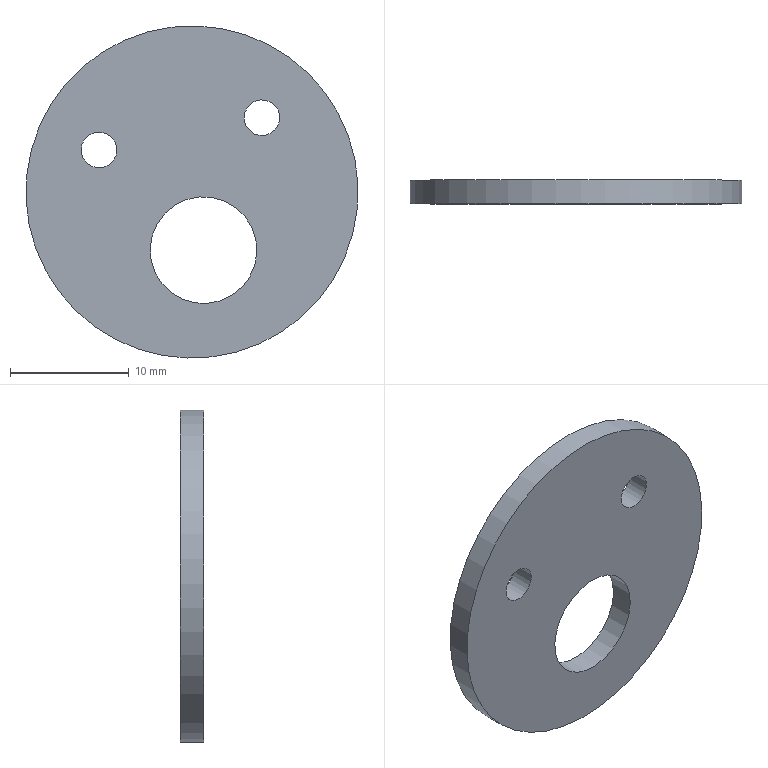Component | NX | ECCENTRIC_SIDE_PLATE_2 | 1 solid | 6 faces | box 28 x 2 x 28 mm | volume 1076 mm3 | cylinder 4 | plane 2 | commonest cylinder face diameters 3 x2 28 x1 9 x1
STEP:
#1=CARTESIAN_POINT('',(0.,0.,0.));
#2=DIRECTION('',(0.,0.,1.));
#3=DIRECTION('',(1.,0.,0.));
#4=AXIS2_PLACEMENT_3D('',#1,#2,#3);
#5=CARTESIAN_POINT('',(49.953,-62.5,29.378));
#6=VERTEX_POINT('',#5);
#7=CARTESIAN_POINT('',(51.424,-62.5,29.669));
#8=DIRECTION('',(0.,1.,0.));
#9=DIRECTION('',(-0.9809,0.,-0.1943));
#10=AXIS2_PLACEMENT_3D('',#7,#8,#9);
#11=CIRCLE('',#10,1.5);
#12=CARTESIAN_POINT('',(45.529,-62.5,23.405));
#13=DIRECTION('',(0.,-1.,0.));
#14=DIRECTION('',(-0.9809,0.,-0.1943));
#15=AXIS2_PLACEMENT_3D('',#12,#13,#14);
#16=PLANE('',#15);
#17=CARTESIAN_POINT('',(-5.5,-5.));
#18=CARTESIAN_POINT('',(-5.5,-7.598));
#19=CARTESIAN_POINT('',(-7.75,-6.299));
#20=CARTESIAN_POINT('',(-10.,-5.));
#21=CARTESIAN_POINT('',(-7.75,-3.701));
#22=CARTESIAN_POINT('',(-5.5,-2.402));
#23=CARTESIAN_POINT('',(-5.5,-5.));
#24=(BOUNDED_CURVE()B_SPLINE_CURVE(2,(#17,#18,#19,#20,#21,#22,#23),.UNSPECIFIED.,.T.,.F.)B_SPLINE_CURVE_WITH_KNOTS((1,2,2,2,2,1),(-2.094,0.,2.094,4.189,6.283,8.378),.UNSPECIFIED.)CURVE()GEOMETRIC_REPRESENTATION_ITEM()RATIONAL_B_SPLINE_CURVE((1.,0.5,1.,0.5,1.,0.5,1.))REPRESENTATION_ITEM(''));
#25=(GEOMETRIC_REPRESENTATION_CONTEXT(2)PARAMETRIC_REPRESENTATION_CONTEXT()REPRESENTATION_CONTEXT('',''));
#26=DEFINITIONAL_REPRESENTATION('',(#24),#25);
#27=PCURVE('',#16,#26);
#28=CARTESIAN_POINT('',(51.424,-42.5,29.669));
#29=DIRECTION('',(0.,-1.,0.));
#30=DIRECTION('',(-0.9809,0.,-0.1943));
#31=AXIS2_PLACEMENT_3D('',#28,#29,#30);
#32=CYLINDRICAL_SURFACE('',#31,1.5);
#33=CARTESIAN_POINT('',(6.283,20.));
#34=DIRECTION('',(-1.,0.));
#35=VECTOR('',#34,1.);
#36=LINE('',#33,#35);
#37=(GEOMETRIC_REPRESENTATION_CONTEXT(2)PARAMETRIC_REPRESENTATION_CONTEXT()REPRESENTATION_CONTEXT('',''));
#38=DEFINITIONAL_REPRESENTATION('',(#36),#37);
#39=PCURVE('',#32,#38);
#40=SURFACE_CURVE('',#11,(#27,#39),.PCURVE_S1.);
#41=EDGE_CURVE('',#6,#6,#40,.T.);
#42=ORIENTED_EDGE('',*,*,#41,.T.);
#43=EDGE_LOOP('',(#42));
#44=FACE_BOUND('',#43,.T.);
#45=CARTESIAN_POINT('',(42.086,-62.5,17.626));
#46=VERTEX_POINT('',#45);
#47=CARTESIAN_POINT('',(46.5,-62.5,18.5));
#48=DIRECTION('',(0.,1.,0.));
#49=DIRECTION('',(-0.9809,0.,-0.1943));
#50=AXIS2_PLACEMENT_3D('',#47,#48,#49);
#51=CIRCLE('',#50,4.5);
#52=CARTESIAN_POINT('',(4.5,5.));
#53=CARTESIAN_POINT('',(4.5,-2.794));
#54=CARTESIAN_POINT('',(-2.25,1.103));
#55=CARTESIAN_POINT('',(-9.,5.));
#56=CARTESIAN_POINT('',(-2.25,8.897));
#57=CARTESIAN_POINT('',(4.5,12.794));
#58=CARTESIAN_POINT('',(4.5,5.));
#59=(BOUNDED_CURVE()B_SPLINE_CURVE(2,(#52,#53,#54,#55,#56,#57,#58),.UNSPECIFIED.,.T.,.F.)B_SPLINE_CURVE_WITH_KNOTS((1,2,2,2,2,1),(-2.094,0.,2.094,4.189,6.283,8.378),.UNSPECIFIED.)CURVE()GEOMETRIC_REPRESENTATION_ITEM()RATIONAL_B_SPLINE_CURVE((1.,0.5,1.,0.5,1.,0.5,1.))REPRESENTATION_ITEM(''));
#60=(GEOMETRIC_REPRESENTATION_CONTEXT(2)PARAMETRIC_REPRESENTATION_CONTEXT()REPRESENTATION_CONTEXT('',''));
#61=DEFINITIONAL_REPRESENTATION('',(#59),#60);
#62=PCURVE('',#16,#61);
#63=CARTESIAN_POINT('',(46.5,-42.5,18.5));
#64=DIRECTION('',(0.,-1.,0.));
#65=DIRECTION('',(-0.9809,0.,-0.1943));
#66=AXIS2_PLACEMENT_3D('',#63,#64,#65);
#67=CYLINDRICAL_SURFACE('',#66,4.5);
#68=CARTESIAN_POINT('',(6.283,20.));
#69=DIRECTION('',(-1.,0.));
#70=VECTOR('',#69,1.);
#71=LINE('',#68,#70);
#72=(GEOMETRIC_REPRESENTATION_CONTEXT(2)PARAMETRIC_REPRESENTATION_CONTEXT()REPRESENTATION_CONTEXT('',''));
#73=DEFINITIONAL_REPRESENTATION('',(#71),#72);
#74=PCURVE('',#67,#73);
#75=SURFACE_CURVE('',#51,(#62,#74),.PCURVE_S1.);
#76=EDGE_CURVE('',#46,#46,#75,.T.);
#77=ORIENTED_EDGE('',*,*,#76,.T.);
#78=EDGE_LOOP('',(#77));
#79=FACE_BOUND('',#78,.T.);
#80=CARTESIAN_POINT('',(31.795,-62.5,20.685));
#81=VERTEX_POINT('',#80);
#82=CARTESIAN_POINT('',(45.529,-62.5,23.405));
#83=DIRECTION('',(0.,1.,0.));
#84=DIRECTION('',(-0.9809,0.,-0.1943));
#85=AXIS2_PLACEMENT_3D('',#82,#83,#84);
#86=CIRCLE('',#85,14.);
#87=CARTESIAN_POINT('',(14.,0.));
#88=CARTESIAN_POINT('',(14.,-24.249));
#89=CARTESIAN_POINT('',(-7.,-12.124));
#90=CARTESIAN_POINT('',(-28.,-0.));
#91=CARTESIAN_POINT('',(-7.,12.124));
#92=CARTESIAN_POINT('',(14.,24.249));
#93=CARTESIAN_POINT('',(14.,0.));
#94=(BOUNDED_CURVE()B_SPLINE_CURVE(2,(#87,#88,#89,#90,#91,#92,#93),.UNSPECIFIED.,.T.,.F.)B_SPLINE_CURVE_WITH_KNOTS((1,2,2,2,2,1),(-2.094,0.,2.094,4.189,6.283,8.378),.UNSPECIFIED.)CURVE()GEOMETRIC_REPRESENTATION_ITEM()RATIONAL_B_SPLINE_CURVE((1.,0.5,1.,0.5,1.,0.5,1.))REPRESENTATION_ITEM(''));
#95=(GEOMETRIC_REPRESENTATION_CONTEXT(2)PARAMETRIC_REPRESENTATION_CONTEXT()REPRESENTATION_CONTEXT('',''));
#96=DEFINITIONAL_REPRESENTATION('',(#94),#95);
#97=PCURVE('',#16,#96);
#98=CARTESIAN_POINT('',(45.529,-60.5,23.405));
#99=DIRECTION('',(0.,-1.,0.));
#100=DIRECTION('',(-0.9809,0.,-0.1943));
#101=AXIS2_PLACEMENT_3D('',#98,#99,#100);
#102=CYLINDRICAL_SURFACE('',#101,14.);
#103=CARTESIAN_POINT('',(6.283,2.));
#104=DIRECTION('',(-1.,0.));
#105=VECTOR('',#104,1.);
#106=LINE('',#103,#105);
#107=(GEOMETRIC_REPRESENTATION_CONTEXT(2)PARAMETRIC_REPRESENTATION_CONTEXT()REPRESENTATION_CONTEXT('',''));
#108=DEFINITIONAL_REPRESENTATION('',(#106),#107);
#109=PCURVE('',#102,#108);
#110=SURFACE_CURVE('',#86,(#97,#109),.PCURVE_S1.);
#111=EDGE_CURVE('',#81,#81,#110,.T.);
#112=ORIENTED_EDGE('',*,*,#111,.F.);
#113=EDGE_LOOP('',(#112));
#114=FACE_BOUND('',#113,.T.);
#115=CARTESIAN_POINT('',(39.162,-62.5,27.241));
#116=VERTEX_POINT('',#115);
#117=CARTESIAN_POINT('',(37.691,-62.5,26.95));
#118=DIRECTION('',(0.,-1.,0.));
#119=DIRECTION('',(0.9809,0.,0.1943));
#120=AXIS2_PLACEMENT_3D('',#117,#118,#119);
#121=CIRCLE('',#120,1.5);
#122=CARTESIAN_POINT('',(7.,-5.));
#123=DIRECTION('',(-1.,0.));
#124=AXIS2_PLACEMENT_2D('',#122,#123);
#125=CIRCLE('',#124,1.5);
#126=(GEOMETRIC_REPRESENTATION_CONTEXT(2)PARAMETRIC_REPRESENTATION_CONTEXT()REPRESENTATION_CONTEXT('',''));
#127=DEFINITIONAL_REPRESENTATION('',(#125),#126);
#128=PCURVE('',#16,#127);
#129=CARTESIAN_POINT('',(37.691,-42.5,26.95));
#130=DIRECTION('',(0.,-1.,0.));
#131=DIRECTION('',(-0.9809,0.,-0.1943));
#132=AXIS2_PLACEMENT_3D('',#129,#130,#131);
#133=CYLINDRICAL_SURFACE('',#132,1.5);
#134=CARTESIAN_POINT('',(3.142,20.));
#135=DIRECTION('',(1.,0.));
#136=VECTOR('',#135,1.);
#137=LINE('',#134,#136);
#138=(GEOMETRIC_REPRESENTATION_CONTEXT(2)PARAMETRIC_REPRESENTATION_CONTEXT()REPRESENTATION_CONTEXT('',''));
#139=DEFINITIONAL_REPRESENTATION('',(#137),#138);
#140=PCURVE('',#133,#139);
#141=SURFACE_CURVE('',#121,(#128,#140),.PCURVE_S1.);
#142=EDGE_CURVE('',#116,#116,#141,.T.);
#143=ORIENTED_EDGE('',*,*,#142,.F.);
#144=EDGE_LOOP('',(#143));
#145=FACE_BOUND('',#144,.T.);
#146=ADVANCED_FACE('',(#44,#79,#114,#145),#16,.T.);
#147=CARTESIAN_POINT('',(52.895,-60.5,29.961));
#148=VERTEX_POINT('',#147);
#149=CARTESIAN_POINT('',(49.953,-60.5,29.378));
#150=VERTEX_POINT('',#149);
#151=CARTESIAN_POINT('',(51.424,-60.5,29.669));
#152=DIRECTION('',(0.,-1.,0.));
#153=DIRECTION('',(0.9809,0.,0.1943));
#154=AXIS2_PLACEMENT_3D('',#151,#152,#153);
#155=CIRCLE('',#154,1.5);
#156=CARTESIAN_POINT('',(45.529,-60.5,23.405));
#157=DIRECTION('',(0.,1.,0.));
#158=DIRECTION('',(0.9809,0.,0.1943));
#159=AXIS2_PLACEMENT_3D('',#156,#157,#158);
#160=PLANE('',#159);
#161=CARTESIAN_POINT('',(8.5,-5.));
#162=CARTESIAN_POINT('',(8.5,-7.598));
#163=CARTESIAN_POINT('',(6.25,-6.299));
#164=CARTESIAN_POINT('',(4.,-5.));
#165=CARTESIAN_POINT('',(6.25,-3.701));
#166=CARTESIAN_POINT('',(8.5,-2.402));
#167=CARTESIAN_POINT('',(8.5,-5.));
#168=(BOUNDED_CURVE()B_SPLINE_CURVE(2,(#161,#162,#163,#164,#165,#166,#167),.UNSPECIFIED.,.T.,.F.)B_SPLINE_CURVE_WITH_KNOTS((1,2,2,2,2,1),(-2.094,0.,2.094,4.189,6.283,8.378),.UNSPECIFIED.)CURVE()GEOMETRIC_REPRESENTATION_ITEM()RATIONAL_B_SPLINE_CURVE((1.,0.5,1.,0.5,1.,0.5,1.))REPRESENTATION_ITEM(''));
#169=(GEOMETRIC_REPRESENTATION_CONTEXT(2)PARAMETRIC_REPRESENTATION_CONTEXT()REPRESENTATION_CONTEXT('',''));
#170=DEFINITIONAL_REPRESENTATION('',(#168),#169);
#171=PCURVE('',#160,#170);
#172=CARTESIAN_POINT('',(3.142,18.));
#173=DIRECTION('',(1.,0.));
#174=VECTOR('',#173,1.);
#175=LINE('',#172,#174);
#176=(GEOMETRIC_REPRESENTATION_CONTEXT(2)PARAMETRIC_REPRESENTATION_CONTEXT()REPRESENTATION_CONTEXT('',''));
#177=DEFINITIONAL_REPRESENTATION('',(#175),#176);
#178=PCURVE('',#32,#177);
#179=SURFACE_CURVE('',#155,(#171,#178),.PCURVE_S1.);
#180=EDGE_CURVE('',#148,#150,#179,.T.);
#181=ORIENTED_EDGE('',*,*,#180,.T.);
#182=CARTESIAN_POINT('',(51.424,-60.5,29.669));
#183=DIRECTION('',(0.,-1.,0.));
#184=DIRECTION('',(0.9809,0.,0.1943));
#185=AXIS2_PLACEMENT_3D('',#182,#183,#184);
#186=CIRCLE('',#185,1.5);
#187=CARTESIAN_POINT('',(8.5,-5.));
#188=CARTESIAN_POINT('',(8.5,-7.598));
#189=CARTESIAN_POINT('',(6.25,-6.299));
#190=CARTESIAN_POINT('',(4.,-5.));
#191=CARTESIAN_POINT('',(6.25,-3.701));
#192=CARTESIAN_POINT('',(8.5,-2.402));
#193=CARTESIAN_POINT('',(8.5,-5.));
#194=(BOUNDED_CURVE()B_SPLINE_CURVE(2,(#187,#188,#189,#190,#191,#192,#193),.UNSPECIFIED.,.T.,.F.)B_SPLINE_CURVE_WITH_KNOTS((1,2,2,2,2,1),(-2.094,0.,2.094,4.189,6.283,8.378),.UNSPECIFIED.)CURVE()GEOMETRIC_REPRESENTATION_ITEM()RATIONAL_B_SPLINE_CURVE((1.,0.5,1.,0.5,1.,0.5,1.))REPRESENTATION_ITEM(''));
#195=(GEOMETRIC_REPRESENTATION_CONTEXT(2)PARAMETRIC_REPRESENTATION_CONTEXT()REPRESENTATION_CONTEXT('',''));
#196=DEFINITIONAL_REPRESENTATION('',(#194),#195);
#197=PCURVE('',#160,#196);
#198=CARTESIAN_POINT('',(-3.142,18.));
#199=DIRECTION('',(1.,0.));
#200=VECTOR('',#199,1.);
#201=LINE('',#198,#200);
#202=(GEOMETRIC_REPRESENTATION_CONTEXT(2)PARAMETRIC_REPRESENTATION_CONTEXT()REPRESENTATION_CONTEXT('',''));
#203=DEFINITIONAL_REPRESENTATION('',(#201),#202);
#204=PCURVE('',#32,#203);
#205=SURFACE_CURVE('',#186,(#197,#204),.PCURVE_S1.);
#206=EDGE_CURVE('',#150,#148,#205,.T.);
#207=ORIENTED_EDGE('',*,*,#206,.T.);
#208=EDGE_LOOP('',(#181,#207));
#209=FACE_BOUND('',#208,.T.);
#210=CARTESIAN_POINT('',(50.914,-60.5,19.374));
#211=VERTEX_POINT('',#210);
#212=CARTESIAN_POINT('',(42.086,-60.5,17.626));
#213=VERTEX_POINT('',#212);
#214=CARTESIAN_POINT('',(46.5,-60.5,18.5));
#215=DIRECTION('',(0.,-1.,0.));
#216=DIRECTION('',(0.9809,0.,0.1943));
#217=AXIS2_PLACEMENT_3D('',#214,#215,#216);
#218=CIRCLE('',#217,4.5);
#219=CARTESIAN_POINT('',(4.5,5.));
#220=CARTESIAN_POINT('',(4.5,-2.794));
#221=CARTESIAN_POINT('',(-2.25,1.103));
#222=CARTESIAN_POINT('',(-9.,5.));
#223=CARTESIAN_POINT('',(-2.25,8.897));
#224=CARTESIAN_POINT('',(4.5,12.794));
#225=CARTESIAN_POINT('',(4.5,5.));
#226=(BOUNDED_CURVE()B_SPLINE_CURVE(2,(#219,#220,#221,#222,#223,#224,#225),.UNSPECIFIED.,.T.,.F.)B_SPLINE_CURVE_WITH_KNOTS((1,2,2,2,2,1),(-2.094,0.,2.094,4.189,6.283,8.378),.UNSPECIFIED.)CURVE()GEOMETRIC_REPRESENTATION_ITEM()RATIONAL_B_SPLINE_CURVE((1.,0.5,1.,0.5,1.,0.5,1.))REPRESENTATION_ITEM(''));
#227=(GEOMETRIC_REPRESENTATION_CONTEXT(2)PARAMETRIC_REPRESENTATION_CONTEXT()REPRESENTATION_CONTEXT('',''));
#228=DEFINITIONAL_REPRESENTATION('',(#226),#227);
#229=PCURVE('',#160,#228);
#230=CARTESIAN_POINT('',(3.142,18.));
#231=DIRECTION('',(1.,0.));
#232=VECTOR('',#231,1.);
#233=LINE('',#230,#232);
#234=(GEOMETRIC_REPRESENTATION_CONTEXT(2)PARAMETRIC_REPRESENTATION_CONTEXT()REPRESENTATION_CONTEXT('',''));
#235=DEFINITIONAL_REPRESENTATION('',(#233),#234);
#236=PCURVE('',#67,#235);
#237=SURFACE_CURVE('',#218,(#229,#236),.PCURVE_S1.);
#238=EDGE_CURVE('',#211,#213,#237,.T.);
#239=ORIENTED_EDGE('',*,*,#238,.T.);
#240=CARTESIAN_POINT('',(46.5,-60.5,18.5));
#241=DIRECTION('',(0.,-1.,0.));
#242=DIRECTION('',(0.9809,0.,0.1943));
#243=AXIS2_PLACEMENT_3D('',#240,#241,#242);
#244=CIRCLE('',#243,4.5);
#245=CARTESIAN_POINT('',(4.5,5.));
#246=CARTESIAN_POINT('',(4.5,-2.794));
#247=CARTESIAN_POINT('',(-2.25,1.103));
#248=CARTESIAN_POINT('',(-9.,5.));
#249=CARTESIAN_POINT('',(-2.25,8.897));
#250=CARTESIAN_POINT('',(4.5,12.794));
#251=CARTESIAN_POINT('',(4.5,5.));
#252=(BOUNDED_CURVE()B_SPLINE_CURVE(2,(#245,#246,#247,#248,#249,#250,#251),.UNSPECIFIED.,.T.,.F.)B_SPLINE_CURVE_WITH_KNOTS((1,2,2,2,2,1),(-2.094,0.,2.094,4.189,6.283,8.378),.UNSPECIFIED.)CURVE()GEOMETRIC_REPRESENTATION_ITEM()RATIONAL_B_SPLINE_CURVE((1.,0.5,1.,0.5,1.,0.5,1.))REPRESENTATION_ITEM(''));
#253=(GEOMETRIC_REPRESENTATION_CONTEXT(2)PARAMETRIC_REPRESENTATION_CONTEXT()REPRESENTATION_CONTEXT('',''));
#254=DEFINITIONAL_REPRESENTATION('',(#252),#253);
#255=PCURVE('',#160,#254);
#256=CARTESIAN_POINT('',(-3.142,18.));
#257=DIRECTION('',(1.,0.));
#258=VECTOR('',#257,1.);
#259=LINE('',#256,#258);
#260=(GEOMETRIC_REPRESENTATION_CONTEXT(2)PARAMETRIC_REPRESENTATION_CONTEXT()REPRESENTATION_CONTEXT('',''));
#261=DEFINITIONAL_REPRESENTATION('',(#259),#260);
#262=PCURVE('',#67,#261);
#263=SURFACE_CURVE('',#244,(#255,#262),.PCURVE_S1.);
#264=EDGE_CURVE('',#213,#211,#263,.T.);
#265=ORIENTED_EDGE('',*,*,#264,.T.);
#266=EDGE_LOOP('',(#239,#265));
#267=FACE_BOUND('',#266,.T.);
#268=CARTESIAN_POINT('',(31.795,-60.5,20.685));
#269=VERTEX_POINT('',#268);
#270=CARTESIAN_POINT('',(45.529,-60.5,23.405));
#271=DIRECTION('',(0.,-1.,0.));
#272=DIRECTION('',(-0.9809,0.,-0.1943));
#273=AXIS2_PLACEMENT_3D('',#270,#271,#272);
#274=CIRCLE('',#273,14.);
#275=CARTESIAN_POINT('',(-14.,0.));
#276=CARTESIAN_POINT('',(-14.,24.249));
#277=CARTESIAN_POINT('',(7.,12.124));
#278=CARTESIAN_POINT('',(28.,0.));
#279=CARTESIAN_POINT('',(7.,-12.124));
#280=CARTESIAN_POINT('',(-14.,-24.249));
#281=CARTESIAN_POINT('',(-14.,0.));
#282=(BOUNDED_CURVE()B_SPLINE_CURVE(2,(#275,#276,#277,#278,#279,#280,#281),.UNSPECIFIED.,.T.,.F.)B_SPLINE_CURVE_WITH_KNOTS((1,2,2,2,2,1),(-2.094,0.,2.094,4.189,6.283,8.378),.UNSPECIFIED.)CURVE()GEOMETRIC_REPRESENTATION_ITEM()RATIONAL_B_SPLINE_CURVE((1.,0.5,1.,0.5,1.,0.5,1.))REPRESENTATION_ITEM(''));
#283=(GEOMETRIC_REPRESENTATION_CONTEXT(2)PARAMETRIC_REPRESENTATION_CONTEXT()REPRESENTATION_CONTEXT('',''));
#284=DEFINITIONAL_REPRESENTATION('',(#282),#283);
#285=PCURVE('',#160,#284);
#286=CARTESIAN_POINT('',(0.,0.));
#287=DIRECTION('',(1.,0.));
#288=VECTOR('',#287,1.);
#289=LINE('',#286,#288);
#290=(GEOMETRIC_REPRESENTATION_CONTEXT(2)PARAMETRIC_REPRESENTATION_CONTEXT()REPRESENTATION_CONTEXT('',''));
#291=DEFINITIONAL_REPRESENTATION('',(#289),#290);
#292=PCURVE('',#102,#291);
#293=SURFACE_CURVE('',#274,(#285,#292),.PCURVE_S1.);
#294=EDGE_CURVE('',#269,#269,#293,.T.);
#295=ORIENTED_EDGE('',*,*,#294,.F.);
#296=EDGE_LOOP('',(#295));
#297=FACE_BOUND('',#296,.T.);
#298=CARTESIAN_POINT('',(39.162,-60.5,27.241));
#299=VERTEX_POINT('',#298);
#300=CARTESIAN_POINT('',(37.691,-60.5,26.95));
#301=DIRECTION('',(0.,1.,0.));
#302=DIRECTION('',(0.9809,0.,0.1943));
#303=AXIS2_PLACEMENT_3D('',#300,#301,#302);
#304=CIRCLE('',#303,1.5);
#305=CARTESIAN_POINT('',(-7.,-5.));
#306=DIRECTION('',(1.,0.));
#307=AXIS2_PLACEMENT_2D('',#305,#306);
#308=CIRCLE('',#307,1.5);
#309=(GEOMETRIC_REPRESENTATION_CONTEXT(2)PARAMETRIC_REPRESENTATION_CONTEXT()REPRESENTATION_CONTEXT('',''));
#310=DEFINITIONAL_REPRESENTATION('',(#308),#309);
#311=PCURVE('',#160,#310);
#312=CARTESIAN_POINT('',(9.425,18.));
#313=DIRECTION('',(-1.,0.));
#314=VECTOR('',#313,1.);
#315=LINE('',#312,#314);
#316=(GEOMETRIC_REPRESENTATION_CONTEXT(2)PARAMETRIC_REPRESENTATION_CONTEXT()REPRESENTATION_CONTEXT('',''));
#317=DEFINITIONAL_REPRESENTATION('',(#315),#316);
#318=PCURVE('',#133,#317);
#319=SURFACE_CURVE('',#304,(#311,#318),.PCURVE_S1.);
#320=EDGE_CURVE('',#299,#299,#319,.T.);
#321=ORIENTED_EDGE('',*,*,#320,.F.);
#322=EDGE_LOOP('',(#321));
#323=FACE_BOUND('',#322,.T.);
#324=ADVANCED_FACE('',(#209,#267,#297,#323),#160,.T.);
#325=ORIENTED_EDGE('',*,*,#111,.T.);
#326=CARTESIAN_POINT('',(31.795,-60.5,20.685));
#327=CARTESIAN_POINT('',(31.795,-62.5,20.685));
#328=B_SPLINE_CURVE_WITH_KNOTS('',1,(#326,#327),.UNSPECIFIED.,.F.,.F.,(2,2),(0.,2.),.PIECEWISE_BEZIER_KNOTS.);
#329=CARTESIAN_POINT('',(0.,0.));
#330=DIRECTION('',(0.,1.));
#331=VECTOR('',#330,1.);
#332=LINE('',#329,#331);
#333=(GEOMETRIC_REPRESENTATION_CONTEXT(2)PARAMETRIC_REPRESENTATION_CONTEXT()REPRESENTATION_CONTEXT('',''));
#334=DEFINITIONAL_REPRESENTATION('',(#332),#333);
#335=PCURVE('',#102,#334);
#336=CARTESIAN_POINT('',(6.283,0.));
#337=DIRECTION('',(0.,1.));
#338=VECTOR('',#337,1.);
#339=LINE('',#336,#338);
#340=(GEOMETRIC_REPRESENTATION_CONTEXT(2)PARAMETRIC_REPRESENTATION_CONTEXT()REPRESENTATION_CONTEXT('',''));
#341=DEFINITIONAL_REPRESENTATION('',(#339),#340);
#342=PCURVE('',#102,#341);
#343=SEAM_CURVE('',#328,(#335,#342),.PCURVE_S1.);
#344=EDGE_CURVE('',#269,#81,#343,.T.);
#345=ORIENTED_EDGE('',*,*,#344,.F.);
#346=ORIENTED_EDGE('',*,*,#294,.T.);
#347=ORIENTED_EDGE('',*,*,#344,.T.);
#348=EDGE_LOOP('',(#325,#345,#346,#347));
#349=FACE_BOUND('',#348,.T.);
#350=ADVANCED_FACE('',(#349),#102,.T.);
#351=ORIENTED_EDGE('',*,*,#238,.T.);
#352=CARTESIAN_POINT('',(42.086,-60.5,17.626));
#353=CARTESIAN_POINT('',(42.086,-62.5,17.626));
#354=B_SPLINE_CURVE_WITH_KNOTS('',1,(#352,#353),.UNSPECIFIED.,.F.,.F.,(2,2),(18.,20.),.PIECEWISE_BEZIER_KNOTS.);
#355=CARTESIAN_POINT('',(6.283,0.));
#356=DIRECTION('',(0.,1.));
#357=VECTOR('',#356,1.);
#358=LINE('',#355,#357);
#359=(GEOMETRIC_REPRESENTATION_CONTEXT(2)PARAMETRIC_REPRESENTATION_CONTEXT()REPRESENTATION_CONTEXT('',''));
#360=DEFINITIONAL_REPRESENTATION('',(#358),#359);
#361=PCURVE('',#67,#360);
#362=CARTESIAN_POINT('',(0.,0.));
#363=DIRECTION('',(0.,1.));
#364=VECTOR('',#363,1.);
#365=LINE('',#362,#364);
#366=(GEOMETRIC_REPRESENTATION_CONTEXT(2)PARAMETRIC_REPRESENTATION_CONTEXT()REPRESENTATION_CONTEXT('',''));
#367=DEFINITIONAL_REPRESENTATION('',(#365),#366);
#368=PCURVE('',#67,#367);
#369=SEAM_CURVE('',#354,(#361,#368),.PCURVE_S1.);
#370=EDGE_CURVE('',#213,#46,#369,.T.);
#371=ORIENTED_EDGE('',*,*,#370,.T.);
#372=ORIENTED_EDGE('',*,*,#76,.T.);
#373=ORIENTED_EDGE('',*,*,#370,.F.);
#374=ORIENTED_EDGE('',*,*,#264,.T.);
#375=EDGE_LOOP('',(#351,#371,#372,#373,#374));
#376=FACE_BOUND('',#375,.F.);
#377=ADVANCED_FACE('',(#376),#67,.F.);
#378=ORIENTED_EDGE('',*,*,#180,.T.);
#379=CARTESIAN_POINT('',(49.953,-60.5,29.378));
#380=CARTESIAN_POINT('',(49.953,-62.5,29.378));
#381=B_SPLINE_CURVE_WITH_KNOTS('',1,(#379,#380),.UNSPECIFIED.,.F.,.F.,(2,2),(18.,20.),.PIECEWISE_BEZIER_KNOTS.);
#382=CARTESIAN_POINT('',(6.283,0.));
#383=DIRECTION('',(0.,1.));
#384=VECTOR('',#383,1.);
#385=LINE('',#382,#384);
#386=(GEOMETRIC_REPRESENTATION_CONTEXT(2)PARAMETRIC_REPRESENTATION_CONTEXT()REPRESENTATION_CONTEXT('',''));
#387=DEFINITIONAL_REPRESENTATION('',(#385),#386);
#388=PCURVE('',#32,#387);
#389=CARTESIAN_POINT('',(0.,0.));
#390=DIRECTION('',(0.,1.));
#391=VECTOR('',#390,1.);
#392=LINE('',#389,#391);
#393=(GEOMETRIC_REPRESENTATION_CONTEXT(2)PARAMETRIC_REPRESENTATION_CONTEXT()REPRESENTATION_CONTEXT('',''));
#394=DEFINITIONAL_REPRESENTATION('',(#392),#393);
#395=PCURVE('',#32,#394);
#396=SEAM_CURVE('',#381,(#388,#395),.PCURVE_S1.);
#397=EDGE_CURVE('',#150,#6,#396,.T.);
#398=ORIENTED_EDGE('',*,*,#397,.T.);
#399=ORIENTED_EDGE('',*,*,#41,.T.);
#400=ORIENTED_EDGE('',*,*,#397,.F.);
#401=ORIENTED_EDGE('',*,*,#206,.T.);
#402=EDGE_LOOP('',(#378,#398,#399,#400,#401));
#403=FACE_BOUND('',#402,.F.);
#404=ADVANCED_FACE('',(#403),#32,.F.);
#405=ORIENTED_EDGE('',*,*,#320,.F.);
#406=CARTESIAN_POINT('',(39.162,-60.5,27.241));
#407=CARTESIAN_POINT('',(39.162,-62.5,27.241));
#408=B_SPLINE_CURVE_WITH_KNOTS('',1,(#406,#407),.UNSPECIFIED.,.F.,.F.,(2,2),(18.,20.),.PIECEWISE_BEZIER_KNOTS.);
#409=CARTESIAN_POINT('',(9.425,0.));
#410=DIRECTION('',(0.,1.));
#411=VECTOR('',#410,1.);
#412=LINE('',#409,#411);
#413=(GEOMETRIC_REPRESENTATION_CONTEXT(2)PARAMETRIC_REPRESENTATION_CONTEXT()REPRESENTATION_CONTEXT('',''));
#414=DEFINITIONAL_REPRESENTATION('',(#412),#413);
#415=PCURVE('',#133,#414);
#416=CARTESIAN_POINT('',(3.142,0.));
#417=DIRECTION('',(0.,1.));
#418=VECTOR('',#417,1.);
#419=LINE('',#416,#418);
#420=(GEOMETRIC_REPRESENTATION_CONTEXT(2)PARAMETRIC_REPRESENTATION_CONTEXT()REPRESENTATION_CONTEXT('',''));
#421=DEFINITIONAL_REPRESENTATION('',(#419),#420);
#422=PCURVE('',#133,#421);
#423=SEAM_CURVE('',#408,(#415,#422),.PCURVE_S1.);
#424=EDGE_CURVE('',#299,#116,#423,.T.);
#425=ORIENTED_EDGE('',*,*,#424,.T.);
#426=ORIENTED_EDGE('',*,*,#142,.F.);
#427=ORIENTED_EDGE('',*,*,#424,.F.);
#428=EDGE_LOOP('',(#405,#425,#426,#427));
#429=FACE_BOUND('',#428,.F.);
#430=ADVANCED_FACE('',(#429),#133,.F.);
#431=CLOSED_SHELL('',(#146,#324,#350,#377,#404,#430));
#432=MANIFOLD_SOLID_BREP('',#431);
#433=(LENGTH_UNIT()NAMED_UNIT(*)SI_UNIT(.MILLI.,.METRE.));
#434=UNCERTAINTY_MEASURE_WITH_UNIT(LENGTH_MEASURE(0.000005),#433,'','');
#435=(NAMED_UNIT(*)PLANE_ANGLE_UNIT()SI_UNIT($,.RADIAN.));
#436=(NAMED_UNIT(*)SI_UNIT($,.STERADIAN.)SOLID_ANGLE_UNIT());
#437=(GEOMETRIC_REPRESENTATION_CONTEXT(3)GLOBAL_UNCERTAINTY_ASSIGNED_CONTEXT((#434))GLOBAL_UNIT_ASSIGNED_CONTEXT((#433,#435,#436))REPRESENTATION_CONTEXT('',''));
#438=ADVANCED_BREP_SHAPE_REPRESENTATION('',(#4,#432),#437);